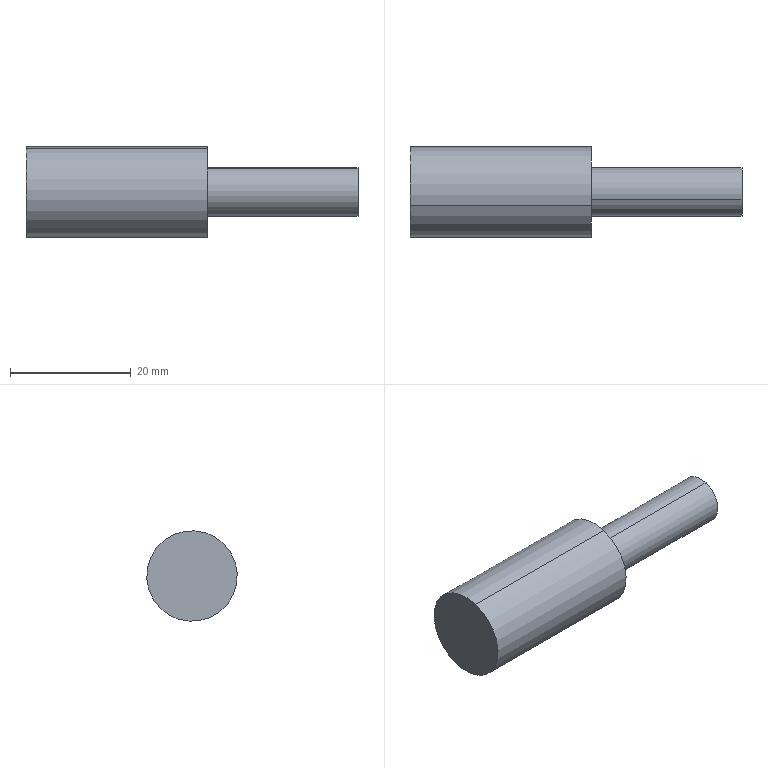Component | SolidWorks | TorqueArmMountingShaft-1-1 | 1 solid | 7 faces | box 55 x 15 x 15 mm | volume 6558 mm3 | cylinder 4 | plane 3 | commonest cylinder face diameters 8 x2 15 x2
build123d program:
from build123d import *

# Parameters (mm, degrees)
SKETCH1_R           = 7.5
BOSS_EXTRUDE1_DEPTH = 15
SKETCH3_R           = 4
BOSS_EXTRUDE3_DEPTH = 25


with BuildPart() as part:
    # Sketch1 → Boss-Extrude1 (new, symmetric)
    with BuildSketch(Plane.XY):
        Circle(SKETCH1_R)
    extrude(amount=BOSS_EXTRUDE1_DEPTH, both=True)

    # Sketch3 → Boss-Extrude3 (add)
    with BuildSketch(Plane.XY.offset(15)):
        Circle(SKETCH3_R)
    extrude(amount=BOSS_EXTRUDE3_DEPTH)


solid = part.part

# Placed as in the assembly
solid = solid.moved(Location((6110.006, 2808.679, 47.375), (0, 90, 0)))
STEP:
#1=COLOUR_RGB('',0.7922,0.8196,0.9333);
#2=FILL_AREA_STYLE_COLOUR('',#1);
#3=FILL_AREA_STYLE('',(#2));
#4=SURFACE_STYLE_FILL_AREA(#3);
#5=SURFACE_SIDE_STYLE('',(#4));
#6=SURFACE_STYLE_USAGE(.BOTH.,#5);
#7=PRESENTATION_STYLE_ASSIGNMENT((#6));
#8=CARTESIAN_POINT('',(242.126,110.626,1.715));
#9=VERTEX_POINT('',#8);
#10=CARTESIAN_POINT('',(242.126,110.53,2.015));
#11=VERTEX_POINT('',#10);
#12=CARTESIAN_POINT('',(242.126,110.578,1.865));
#13=DIRECTION('',(1.,0.,-0.));
#14=DIRECTION('',(0.,0.303,-0.953));
#15=AXIS2_PLACEMENT_3D('',#12,#13,#14);
#16=CIRCLE('',#15,0.1575);
#17=EDGE_CURVE('',#9,#11,#16,.T.);
#18=ORIENTED_EDGE('',*,*,#17,.F.);
#19=CARTESIAN_POINT('',(241.142,110.626,1.715));
#20=VERTEX_POINT('',#19);
#21=CARTESIAN_POINT('',(242.126,110.626,1.715));
#22=DIRECTION('',(-1.,-0.,0.));
#23=VECTOR('',#22,39.37);
#24=LINE('',#21,#23);
#25=EDGE_CURVE('',#9,#20,#24,.T.);
#26=ORIENTED_EDGE('',*,*,#25,.T.);
#27=CARTESIAN_POINT('',(241.142,110.53,2.015));
#28=VERTEX_POINT('',#27);
#29=CARTESIAN_POINT('',(241.142,110.578,1.865));
#30=DIRECTION('',(1.,0.,-0.));
#31=DIRECTION('',(0.,0.303,-0.953));
#32=AXIS2_PLACEMENT_3D('',#29,#30,#31);
#33=CIRCLE('',#32,0.1575);
#34=EDGE_CURVE('',#20,#28,#33,.T.);
#35=ORIENTED_EDGE('',*,*,#34,.T.);
#36=CARTESIAN_POINT('',(242.126,110.53,2.015));
#37=DIRECTION('',(-1.,-0.,0.));
#38=VECTOR('',#37,39.37);
#39=LINE('',#36,#38);
#40=EDGE_CURVE('',#11,#28,#39,.T.);
#41=ORIENTED_EDGE('',*,*,#40,.F.);
#42=EDGE_LOOP('',(#18,#26,#35,#41));
#43=FACE_OUTER_BOUND('',#42,.T.);
#44=CARTESIAN_POINT('',(242.126,110.578,1.865));
#45=DIRECTION('',(-1.,-0.,0.));
#46=DIRECTION('',(0.,-0.303,0.953));
#47=AXIS2_PLACEMENT_3D('',#44,#45,#46);
#48=CYLINDRICAL_SURFACE('',#47,0.1575);
#49=ADVANCED_FACE('',(#43),#48,.T.);
#50=CARTESIAN_POINT('',(241.142,110.667,1.584));
#51=VERTEX_POINT('',#50);
#52=CARTESIAN_POINT('',(241.142,110.488,2.147));
#53=VERTEX_POINT('',#52);
#54=CARTESIAN_POINT('',(241.142,110.578,1.865));
#55=DIRECTION('',(1.,0.,-0.));
#56=DIRECTION('',(0.,0.303,-0.953));
#57=AXIS2_PLACEMENT_3D('',#54,#55,#56);
#58=CIRCLE('',#57,0.2953);
#59=EDGE_CURVE('',#51,#53,#58,.T.);
#60=ORIENTED_EDGE('',*,*,#59,.F.);
#61=CARTESIAN_POINT('',(239.961,110.667,1.584));
#62=VERTEX_POINT('',#61);
#63=CARTESIAN_POINT('',(241.142,110.667,1.584));
#64=DIRECTION('',(-1.,-0.,0.));
#65=VECTOR('',#64,39.37);
#66=LINE('',#63,#65);
#67=EDGE_CURVE('',#51,#62,#66,.T.);
#68=ORIENTED_EDGE('',*,*,#67,.T.);
#69=CARTESIAN_POINT('',(239.961,110.488,2.147));
#70=VERTEX_POINT('',#69);
#71=CARTESIAN_POINT('',(239.961,110.578,1.865));
#72=DIRECTION('',(1.,0.,-0.));
#73=DIRECTION('',(0.,0.303,-0.953));
#74=AXIS2_PLACEMENT_3D('',#71,#72,#73);
#75=CIRCLE('',#74,0.2953);
#76=EDGE_CURVE('',#62,#70,#75,.T.);
#77=ORIENTED_EDGE('',*,*,#76,.T.);
#78=CARTESIAN_POINT('',(241.142,110.488,2.147));
#79=DIRECTION('',(-1.,-0.,0.));
#80=VECTOR('',#79,39.37);
#81=LINE('',#78,#80);
#82=EDGE_CURVE('',#53,#70,#81,.T.);
#83=ORIENTED_EDGE('',*,*,#82,.F.);
#84=EDGE_LOOP('',(#60,#68,#77,#83));
#85=FACE_OUTER_BOUND('',#84,.T.);
#86=CARTESIAN_POINT('',(241.142,110.578,1.865));
#87=DIRECTION('',(-1.,-0.,0.));
#88=DIRECTION('',(0.,-0.303,0.953));
#89=AXIS2_PLACEMENT_3D('',#86,#87,#88);
#90=CYLINDRICAL_SURFACE('',#89,0.2953);
#91=ADVANCED_FACE('',(#85),#90,.T.);
#92=CARTESIAN_POINT('',(241.142,110.578,1.865));
#93=DIRECTION('',(1.,0.,-0.));
#94=DIRECTION('',(0.,0.303,-0.953));
#95=AXIS2_PLACEMENT_3D('',#92,#93,#94);
#96=CIRCLE('',#95,0.2953);
#97=EDGE_CURVE('',#53,#51,#96,.T.);
#98=ORIENTED_EDGE('',*,*,#97,.T.);
#99=ORIENTED_EDGE('',*,*,#59,.T.);
#100=EDGE_LOOP('',(#98,#99));
#101=FACE_OUTER_BOUND('',#100,.T.);
#102=CARTESIAN_POINT('',(241.142,110.578,1.865));
#103=DIRECTION('',(1.,0.,-0.));
#104=DIRECTION('',(0.,0.303,-0.953));
#105=AXIS2_PLACEMENT_3D('',#102,#103,#104);
#106=CIRCLE('',#105,0.1575);
#107=EDGE_CURVE('',#28,#20,#106,.T.);
#108=ORIENTED_EDGE('',*,*,#107,.F.);
#109=ORIENTED_EDGE('',*,*,#34,.F.);
#110=EDGE_LOOP('',(#108,#109));
#111=FACE_BOUND('',#110,.T.);
#112=CARTESIAN_POINT('',(241.142,110.578,1.865));
#113=DIRECTION('',(1.,0.,-0.));
#114=DIRECTION('',(-0.,0.303,-0.953));
#115=AXIS2_PLACEMENT_3D('',#112,#113,#114);
#116=PLANE('',#115);
#117=ADVANCED_FACE('',(#101,#111),#116,.T.);
#118=ORIENTED_EDGE('',*,*,#67,.F.);
#119=ORIENTED_EDGE('',*,*,#97,.F.);
#120=ORIENTED_EDGE('',*,*,#82,.T.);
#121=CARTESIAN_POINT('',(239.961,110.578,1.865));
#122=DIRECTION('',(1.,0.,-0.));
#123=DIRECTION('',(0.,0.303,-0.953));
#124=AXIS2_PLACEMENT_3D('',#121,#122,#123);
#125=CIRCLE('',#124,0.2953);
#126=EDGE_CURVE('',#70,#62,#125,.T.);
#127=ORIENTED_EDGE('',*,*,#126,.T.);
#128=EDGE_LOOP('',(#118,#119,#120,#127));
#129=FACE_OUTER_BOUND('',#128,.T.);
#130=CARTESIAN_POINT('',(241.142,110.578,1.865));
#131=DIRECTION('',(-1.,-0.,0.));
#132=DIRECTION('',(0.,-0.303,0.953));
#133=AXIS2_PLACEMENT_3D('',#130,#131,#132);
#134=CYLINDRICAL_SURFACE('',#133,0.2953);
#135=ADVANCED_FACE('',(#129),#134,.T.);
#136=ORIENTED_EDGE('',*,*,#126,.F.);
#137=ORIENTED_EDGE('',*,*,#76,.F.);
#138=EDGE_LOOP('',(#136,#137));
#139=FACE_OUTER_BOUND('',#138,.T.);
#140=CARTESIAN_POINT('',(239.961,110.578,1.865));
#141=DIRECTION('',(1.,0.,-0.));
#142=DIRECTION('',(-0.,0.303,-0.953));
#143=AXIS2_PLACEMENT_3D('',#140,#141,#142);
#144=PLANE('',#143);
#145=ADVANCED_FACE('',(#139),#144,.F.);
#146=ORIENTED_EDGE('',*,*,#25,.F.);
#147=CARTESIAN_POINT('',(242.126,110.578,1.865));
#148=DIRECTION('',(1.,0.,-0.));
#149=DIRECTION('',(0.,0.303,-0.953));
#150=AXIS2_PLACEMENT_3D('',#147,#148,#149);
#151=CIRCLE('',#150,0.1575);
#152=EDGE_CURVE('',#11,#9,#151,.T.);
#153=ORIENTED_EDGE('',*,*,#152,.F.);
#154=ORIENTED_EDGE('',*,*,#40,.T.);
#155=ORIENTED_EDGE('',*,*,#107,.T.);
#156=EDGE_LOOP('',(#146,#153,#154,#155));
#157=FACE_OUTER_BOUND('',#156,.T.);
#158=CARTESIAN_POINT('',(242.126,110.578,1.865));
#159=DIRECTION('',(-1.,-0.,0.));
#160=DIRECTION('',(0.,-0.303,0.953));
#161=AXIS2_PLACEMENT_3D('',#158,#159,#160);
#162=CYLINDRICAL_SURFACE('',#161,0.1575);
#163=ADVANCED_FACE('',(#157),#162,.T.);
#164=ORIENTED_EDGE('',*,*,#152,.T.);
#165=ORIENTED_EDGE('',*,*,#17,.T.);
#166=EDGE_LOOP('',(#164,#165));
#167=FACE_OUTER_BOUND('',#166,.T.);
#168=CARTESIAN_POINT('',(242.126,110.578,1.865));
#169=DIRECTION('',(1.,0.,-0.));
#170=DIRECTION('',(-0.,0.303,-0.953));
#171=AXIS2_PLACEMENT_3D('',#168,#169,#170);
#172=PLANE('',#171);
#173=ADVANCED_FACE('',(#167),#172,.T.);
#174=CLOSED_SHELL('',(#49,#91,#117,#135,#145,#163,#173));
#175=MANIFOLD_SOLID_BREP('',#174);
#176=STYLED_ITEM('',(#7),#175);
#177=(LENGTH_UNIT()NAMED_UNIT(*)SI_UNIT($,.METRE.));
#178=LENGTH_MEASURE_WITH_UNIT(LENGTH_MEASURE(0.0254),#177);
#179=DIMENSIONAL_EXPONENTS(1.,0.,0.,0.,0.,0.,0.);
#180=(CONVERSION_BASED_UNIT('',#178)LENGTH_UNIT()NAMED_UNIT(#179));
#181=UNCERTAINTY_MEASURE_WITH_UNIT(LENGTH_MEASURE(0.00001),#180,'','');
#182=(NAMED_UNIT(*)PLANE_ANGLE_UNIT()SI_UNIT($,.RADIAN.));
#183=(NAMED_UNIT(*)SI_UNIT($,.STERADIAN.)SOLID_ANGLE_UNIT());
#184=(GEOMETRIC_REPRESENTATION_CONTEXT(3)GLOBAL_UNCERTAINTY_ASSIGNED_CONTEXT((#181))GLOBAL_UNIT_ASSIGNED_CONTEXT((#180,#182,#183))REPRESENTATION_CONTEXT('',''));
#185=MECHANICAL_DESIGN_GEOMETRIC_PRESENTATION_REPRESENTATION('',(#176),#184);
#186=PRESENTATION_LAYER_ASSIGNMENT('','',(#176));
#187=CARTESIAN_POINT('',(0.,0.,0.));
#188=DIRECTION('',(0.,0.,1.));
#189=DIRECTION('',(1.,0.,0.));
#190=AXIS2_PLACEMENT_3D('',#187,#188,#189);
#191=(LENGTH_UNIT()NAMED_UNIT(*)SI_UNIT($,.METRE.));
#192=LENGTH_MEASURE_WITH_UNIT(LENGTH_MEASURE(0.0254),#191);
#193=DIMENSIONAL_EXPONENTS(1.,0.,0.,0.,0.,0.,0.);
#194=(CONVERSION_BASED_UNIT('',#192)LENGTH_UNIT()NAMED_UNIT(#193));
#195=UNCERTAINTY_MEASURE_WITH_UNIT(LENGTH_MEASURE(0.00001),#194,'','');
#196=(NAMED_UNIT(*)PLANE_ANGLE_UNIT()SI_UNIT($,.RADIAN.));
#197=(NAMED_UNIT(*)SI_UNIT($,.STERADIAN.)SOLID_ANGLE_UNIT());
#198=(GEOMETRIC_REPRESENTATION_CONTEXT(3)GLOBAL_UNCERTAINTY_ASSIGNED_CONTEXT((#195))GLOBAL_UNIT_ASSIGNED_CONTEXT((#194,#196,#197))REPRESENTATION_CONTEXT('',''));
#199=ADVANCED_BREP_SHAPE_REPRESENTATION('',(#175,#190),#198);